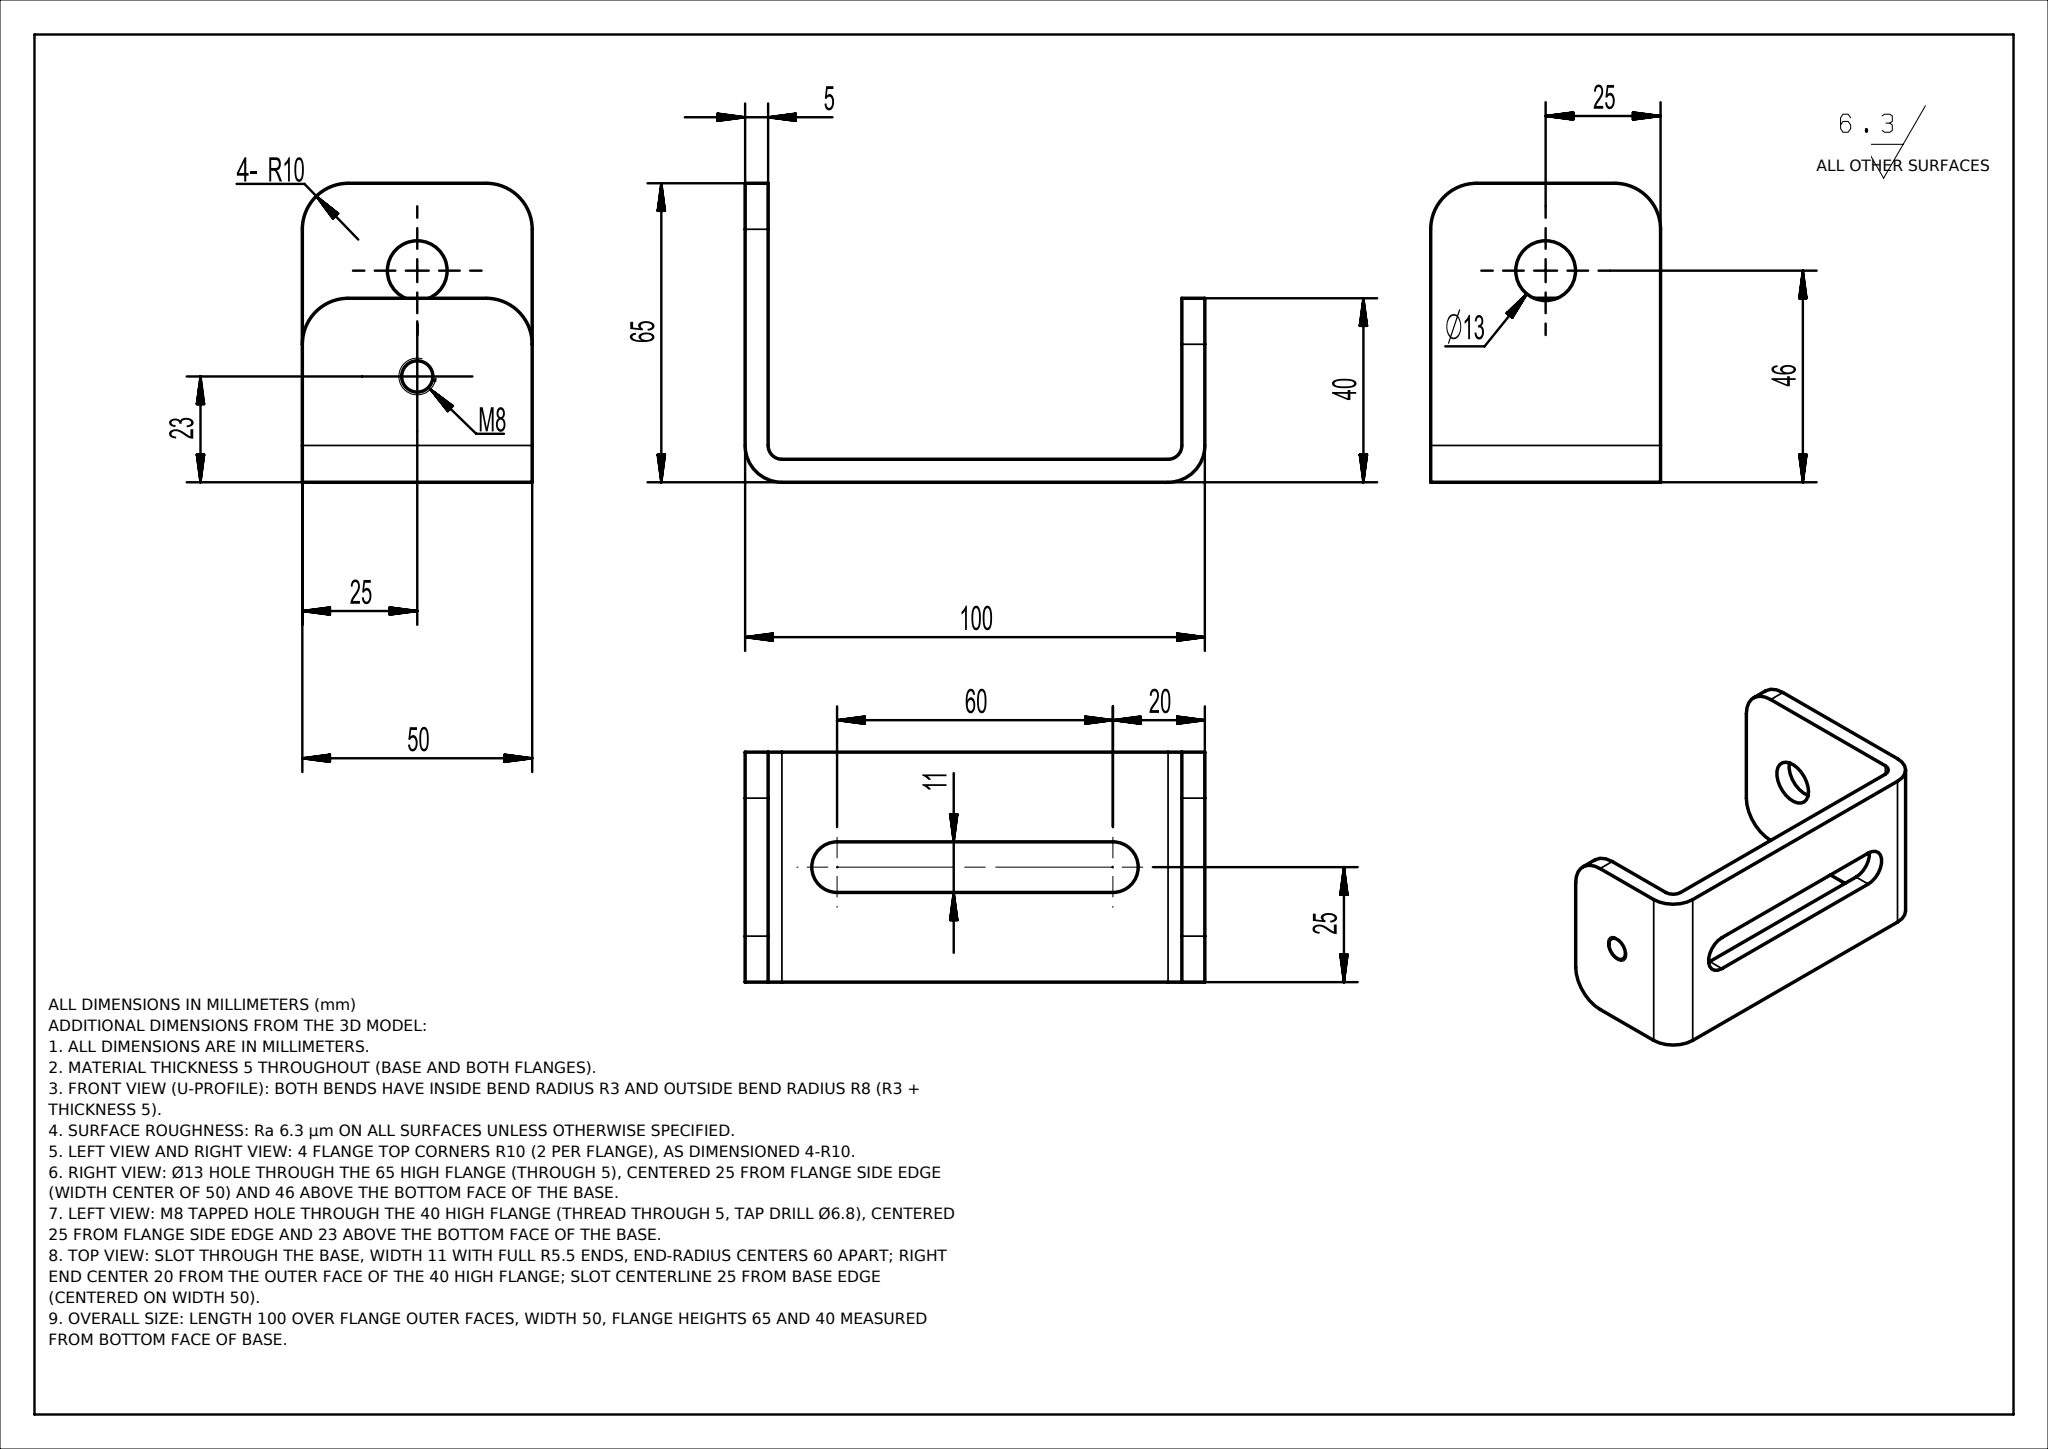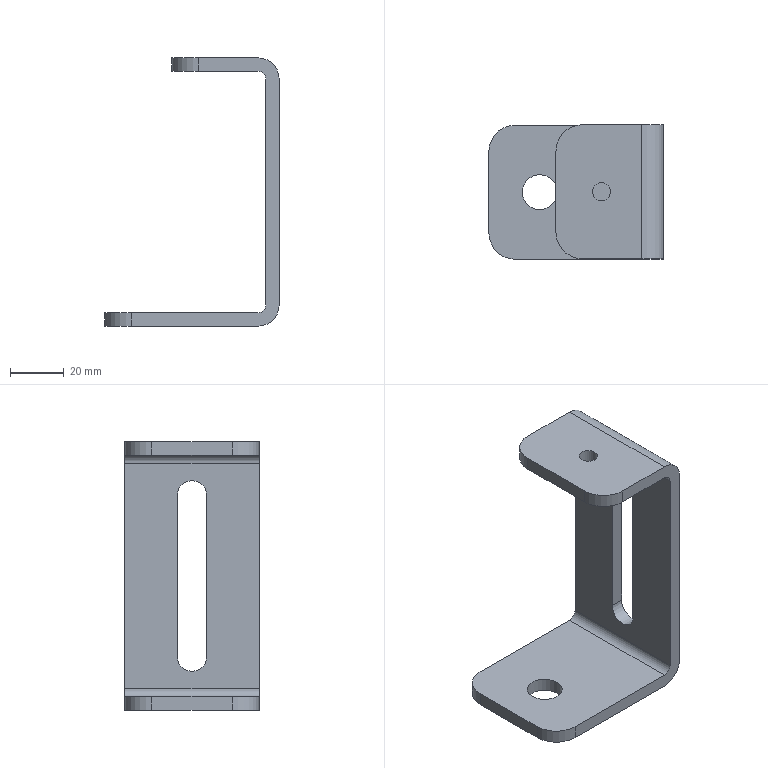Part | NX | mm | 1 solid | 24 faces | box 65 x 50 x 100 mm | volume 42520 mm3 | plane 12 | cylinder 12 | commonest cylinder face diameters 20 x4 6 x2 16 x2 11 x2 6.8 x1 13 x1
STEP:
#1=CARTESIAN_POINT('',(0.,0.,0.));
#2=DIRECTION('',(0.,0.,1.));
#3=DIRECTION('',(1.,0.,0.));
#4=AXIS2_PLACEMENT_3D('',#1,#2,#3);
#5=(LENGTH_UNIT()NAMED_UNIT(*)SI_UNIT(.MILLI.,.METRE.));
#6=UNCERTAINTY_MEASURE_WITH_UNIT(LENGTH_MEASURE(0.00002),#5,'','');
#7=(NAMED_UNIT(*)PLANE_ANGLE_UNIT()SI_UNIT($,.RADIAN.));
#8=PLANE_ANGLE_MEASURE_WITH_UNIT(PLANE_ANGLE_MEASURE(0.01745),#7);
#9=DIMENSIONAL_EXPONENTS(0.,0.,0.,0.,0.,0.,0.);
#10=(CONVERSION_BASED_UNIT('',#8)NAMED_UNIT(#9)PLANE_ANGLE_UNIT());
#11=(NAMED_UNIT(*)SI_UNIT($,.STERADIAN.)SOLID_ANGLE_UNIT());
#12=(GEOMETRIC_REPRESENTATION_CONTEXT(3)GLOBAL_UNCERTAINTY_ASSIGNED_CONTEXT((#6))GLOBAL_UNIT_ASSIGNED_CONTEXT((#5,#10,#11))REPRESENTATION_CONTEXT('',''));
#13=SHAPE_REPRESENTATION('',(#4),#12);
#14=CARTESIAN_POINT('',(10.,0.,5.));
#15=VERTEX_POINT('',#14);
#16=CARTESIAN_POINT('',(57.,0.,5.));
#17=VERTEX_POINT('',#16);
#18=CARTESIAN_POINT('',(0.,0.,5.));
#19=DIRECTION('',(1.,0.,0.));
#20=VECTOR('',#19,1.);
#21=LINE('',#18,#20);
#22=EDGE_CURVE('',#15,#17,#21,.T.);
#23=ORIENTED_EDGE('',*,*,#22,.F.);
#24=CARTESIAN_POINT('',(10.,0.,0.));
#25=VERTEX_POINT('',#24);
#26=CARTESIAN_POINT('',(10.,0.,100.));
#27=DIRECTION('',(0.,0.,-1.));
#28=VECTOR('',#27,1.);
#29=LINE('',#26,#28);
#30=EDGE_CURVE('',#15,#25,#29,.T.);
#31=ORIENTED_EDGE('',*,*,#30,.T.);
#32=CARTESIAN_POINT('',(57.,0.,0.));
#33=VERTEX_POINT('',#32);
#34=CARTESIAN_POINT('',(0.,0.,0.));
#35=DIRECTION('',(1.,0.,0.));
#36=VECTOR('',#35,1.);
#37=LINE('',#34,#36);
#38=EDGE_CURVE('',#25,#33,#37,.T.);
#39=ORIENTED_EDGE('',*,*,#38,.T.);
#40=CARTESIAN_POINT('',(65.,0.,8.));
#41=VERTEX_POINT('',#40);
#42=CARTESIAN_POINT('',(57.,0.,8.));
#43=DIRECTION('',(0.,-1.,0.));
#44=DIRECTION('',(0.,0.,1.));
#45=AXIS2_PLACEMENT_3D('',#42,#43,#44);
#46=CIRCLE('',#45,8.);
#47=EDGE_CURVE('',#33,#41,#46,.T.);
#48=ORIENTED_EDGE('',*,*,#47,.T.);
#49=CARTESIAN_POINT('',(65.,0.,92.));
#50=VERTEX_POINT('',#49);
#51=CARTESIAN_POINT('',(65.,0.,0.));
#52=DIRECTION('',(-0.,0.,1.));
#53=VECTOR('',#52,1.);
#54=LINE('',#51,#53);
#55=EDGE_CURVE('',#41,#50,#54,.T.);
#56=ORIENTED_EDGE('',*,*,#55,.T.);
#57=CARTESIAN_POINT('',(57.,0.,100.));
#58=VERTEX_POINT('',#57);
#59=CARTESIAN_POINT('',(57.,0.,92.));
#60=DIRECTION('',(0.,-1.,0.));
#61=DIRECTION('',(0.,0.,1.));
#62=AXIS2_PLACEMENT_3D('',#59,#60,#61);
#63=CIRCLE('',#62,8.);
#64=EDGE_CURVE('',#50,#58,#63,.T.);
#65=ORIENTED_EDGE('',*,*,#64,.T.);
#66=CARTESIAN_POINT('',(35.,0.,100.));
#67=VERTEX_POINT('',#66);
#68=CARTESIAN_POINT('',(65.,0.,100.));
#69=DIRECTION('',(-1.,0.,0.));
#70=VECTOR('',#69,1.);
#71=LINE('',#68,#70);
#72=EDGE_CURVE('',#58,#67,#71,.T.);
#73=ORIENTED_EDGE('',*,*,#72,.T.);
#74=CARTESIAN_POINT('',(35.,0.,95.));
#75=VERTEX_POINT('',#74);
#76=CARTESIAN_POINT('',(35.,0.,100.));
#77=DIRECTION('',(0.,0.,-1.));
#78=VECTOR('',#77,1.);
#79=LINE('',#76,#78);
#80=EDGE_CURVE('',#67,#75,#79,.T.);
#81=ORIENTED_EDGE('',*,*,#80,.T.);
#82=CARTESIAN_POINT('',(57.,0.,95.));
#83=VERTEX_POINT('',#82);
#84=CARTESIAN_POINT('',(65.,0.,95.));
#85=DIRECTION('',(-1.,0.,0.));
#86=VECTOR('',#85,1.);
#87=LINE('',#84,#86);
#88=EDGE_CURVE('',#83,#75,#87,.T.);
#89=ORIENTED_EDGE('',*,*,#88,.F.);
#90=CARTESIAN_POINT('',(60.,0.,92.));
#91=VERTEX_POINT('',#90);
#92=CARTESIAN_POINT('',(57.,0.,92.));
#93=DIRECTION('',(0.,-1.,0.));
#94=DIRECTION('',(0.,0.,1.));
#95=AXIS2_PLACEMENT_3D('',#92,#93,#94);
#96=CIRCLE('',#95,3.);
#97=EDGE_CURVE('',#91,#83,#96,.T.);
#98=ORIENTED_EDGE('',*,*,#97,.F.);
#99=CARTESIAN_POINT('',(60.,0.,8.));
#100=VERTEX_POINT('',#99);
#101=CARTESIAN_POINT('',(60.,0.,-0.));
#102=DIRECTION('',(-0.,0.,1.));
#103=VECTOR('',#102,1.);
#104=LINE('',#101,#103);
#105=EDGE_CURVE('',#100,#91,#104,.T.);
#106=ORIENTED_EDGE('',*,*,#105,.F.);
#107=CARTESIAN_POINT('',(57.,0.,8.));
#108=DIRECTION('',(0.,-1.,0.));
#109=DIRECTION('',(0.,0.,1.));
#110=AXIS2_PLACEMENT_3D('',#107,#108,#109);
#111=CIRCLE('',#110,3.);
#112=EDGE_CURVE('',#17,#100,#111,.T.);
#113=ORIENTED_EDGE('',*,*,#112,.F.);
#114=EDGE_LOOP('',(#23,#31,#39,#48,#56,#65,#73,#81,#89,#98,#106,#113));
#115=FACE_OUTER_BOUND('',#114,.T.);
#116=CARTESIAN_POINT('',(65.,0.,100.));
#117=DIRECTION('',(0.,-1.,0.));
#118=DIRECTION('',(-1.,0.,0.));
#119=AXIS2_PLACEMENT_3D('',#116,#117,#118);
#120=PLANE('',#119);
#121=ADVANCED_FACE('',(#115),#120,.T.);
#122=CARTESIAN_POINT('',(25.,10.,95.));
#123=VERTEX_POINT('',#122);
#124=CARTESIAN_POINT('',(25.,40.,95.));
#125=VERTEX_POINT('',#124);
#126=CARTESIAN_POINT('',(25.,0.,95.));
#127=DIRECTION('',(0.,1.,0.));
#128=VECTOR('',#127,1.);
#129=LINE('',#126,#128);
#130=EDGE_CURVE('',#123,#125,#129,.T.);
#131=ORIENTED_EDGE('',*,*,#130,.F.);
#132=CARTESIAN_POINT('',(25.,10.,100.));
#133=VERTEX_POINT('',#132);
#134=CARTESIAN_POINT('',(25.,10.,100.));
#135=DIRECTION('',(0.,0.,1.));
#136=VECTOR('',#135,1.);
#137=LINE('',#134,#136);
#138=EDGE_CURVE('',#123,#133,#137,.T.);
#139=ORIENTED_EDGE('',*,*,#138,.T.);
#140=CARTESIAN_POINT('',(25.,40.,100.));
#141=VERTEX_POINT('',#140);
#142=CARTESIAN_POINT('',(25.,0.,100.));
#143=DIRECTION('',(0.,1.,0.));
#144=VECTOR('',#143,1.);
#145=LINE('',#142,#144);
#146=EDGE_CURVE('',#133,#141,#145,.T.);
#147=ORIENTED_EDGE('',*,*,#146,.T.);
#148=CARTESIAN_POINT('',(25.,40.,100.));
#149=DIRECTION('',(0.,0.,-1.));
#150=VECTOR('',#149,1.);
#151=LINE('',#148,#150);
#152=EDGE_CURVE('',#141,#125,#151,.T.);
#153=ORIENTED_EDGE('',*,*,#152,.T.);
#154=EDGE_LOOP('',(#131,#139,#147,#153));
#155=FACE_OUTER_BOUND('',#154,.T.);
#156=CARTESIAN_POINT('',(25.,0.,100.));
#157=DIRECTION('',(-1.,0.,0.));
#158=DIRECTION('',(0.,1.,0.));
#159=AXIS2_PLACEMENT_3D('',#156,#157,#158);
#160=PLANE('',#159);
#161=ADVANCED_FACE('',(#155),#160,.T.);
#162=CARTESIAN_POINT('',(10.,50.,0.));
#163=VERTEX_POINT('',#162);
#164=CARTESIAN_POINT('',(57.,50.,0.));
#165=VERTEX_POINT('',#164);
#166=CARTESIAN_POINT('',(0.,50.,0.));
#167=DIRECTION('',(1.,0.,0.));
#168=VECTOR('',#167,1.);
#169=LINE('',#166,#168);
#170=EDGE_CURVE('',#163,#165,#169,.T.);
#171=ORIENTED_EDGE('',*,*,#170,.F.);
#172=CARTESIAN_POINT('',(10.,50.,5.));
#173=VERTEX_POINT('',#172);
#174=CARTESIAN_POINT('',(10.,50.,0.));
#175=DIRECTION('',(0.,0.,1.));
#176=VECTOR('',#175,1.);
#177=LINE('',#174,#176);
#178=EDGE_CURVE('',#163,#173,#177,.T.);
#179=ORIENTED_EDGE('',*,*,#178,.T.);
#180=CARTESIAN_POINT('',(57.,50.,5.));
#181=VERTEX_POINT('',#180);
#182=CARTESIAN_POINT('',(0.,50.,5.));
#183=DIRECTION('',(1.,0.,0.));
#184=VECTOR('',#183,1.);
#185=LINE('',#182,#184);
#186=EDGE_CURVE('',#173,#181,#185,.T.);
#187=ORIENTED_EDGE('',*,*,#186,.T.);
#188=CARTESIAN_POINT('',(60.,50.,8.));
#189=VERTEX_POINT('',#188);
#190=CARTESIAN_POINT('',(57.,50.,8.));
#191=DIRECTION('',(0.,-1.,0.));
#192=DIRECTION('',(0.,0.,1.));
#193=AXIS2_PLACEMENT_3D('',#190,#191,#192);
#194=CIRCLE('',#193,3.);
#195=EDGE_CURVE('',#181,#189,#194,.T.);
#196=ORIENTED_EDGE('',*,*,#195,.T.);
#197=CARTESIAN_POINT('',(60.,50.,92.));
#198=VERTEX_POINT('',#197);
#199=CARTESIAN_POINT('',(60.,50.,-0.));
#200=DIRECTION('',(-0.,0.,1.));
#201=VECTOR('',#200,1.);
#202=LINE('',#199,#201);
#203=EDGE_CURVE('',#189,#198,#202,.T.);
#204=ORIENTED_EDGE('',*,*,#203,.T.);
#205=CARTESIAN_POINT('',(57.,50.,95.));
#206=VERTEX_POINT('',#205);
#207=CARTESIAN_POINT('',(57.,50.,92.));
#208=DIRECTION('',(0.,-1.,0.));
#209=DIRECTION('',(0.,0.,1.));
#210=AXIS2_PLACEMENT_3D('',#207,#208,#209);
#211=CIRCLE('',#210,3.);
#212=EDGE_CURVE('',#198,#206,#211,.T.);
#213=ORIENTED_EDGE('',*,*,#212,.T.);
#214=CARTESIAN_POINT('',(35.,50.,95.));
#215=VERTEX_POINT('',#214);
#216=CARTESIAN_POINT('',(65.,50.,95.));
#217=DIRECTION('',(-1.,0.,0.));
#218=VECTOR('',#217,1.);
#219=LINE('',#216,#218);
#220=EDGE_CURVE('',#206,#215,#219,.T.);
#221=ORIENTED_EDGE('',*,*,#220,.T.);
#222=CARTESIAN_POINT('',(35.,50.,100.));
#223=VERTEX_POINT('',#222);
#224=CARTESIAN_POINT('',(35.,50.,0.));
#225=DIRECTION('',(0.,0.,1.));
#226=VECTOR('',#225,1.);
#227=LINE('',#224,#226);
#228=EDGE_CURVE('',#215,#223,#227,.T.);
#229=ORIENTED_EDGE('',*,*,#228,.T.);
#230=CARTESIAN_POINT('',(57.,50.,100.));
#231=VERTEX_POINT('',#230);
#232=CARTESIAN_POINT('',(65.,50.,100.));
#233=DIRECTION('',(-1.,0.,0.));
#234=VECTOR('',#233,1.);
#235=LINE('',#232,#234);
#236=EDGE_CURVE('',#231,#223,#235,.T.);
#237=ORIENTED_EDGE('',*,*,#236,.F.);
#238=CARTESIAN_POINT('',(65.,50.,92.));
#239=VERTEX_POINT('',#238);
#240=CARTESIAN_POINT('',(57.,50.,92.));
#241=DIRECTION('',(0.,-1.,0.));
#242=DIRECTION('',(0.,0.,1.));
#243=AXIS2_PLACEMENT_3D('',#240,#241,#242);
#244=CIRCLE('',#243,8.);
#245=EDGE_CURVE('',#239,#231,#244,.T.);
#246=ORIENTED_EDGE('',*,*,#245,.F.);
#247=CARTESIAN_POINT('',(65.,50.,8.));
#248=VERTEX_POINT('',#247);
#249=CARTESIAN_POINT('',(65.,50.,0.));
#250=DIRECTION('',(-0.,0.,1.));
#251=VECTOR('',#250,1.);
#252=LINE('',#249,#251);
#253=EDGE_CURVE('',#248,#239,#252,.T.);
#254=ORIENTED_EDGE('',*,*,#253,.F.);
#255=CARTESIAN_POINT('',(57.,50.,8.));
#256=DIRECTION('',(0.,-1.,0.));
#257=DIRECTION('',(0.,0.,1.));
#258=AXIS2_PLACEMENT_3D('',#255,#256,#257);
#259=CIRCLE('',#258,8.);
#260=EDGE_CURVE('',#165,#248,#259,.T.);
#261=ORIENTED_EDGE('',*,*,#260,.F.);
#262=EDGE_LOOP('',(#171,#179,#187,#196,#204,#213,#221,#229,#237,#246,#254,#261));
#263=FACE_OUTER_BOUND('',#262,.T.);
#264=CARTESIAN_POINT('',(0.,50.,0.));
#265=DIRECTION('',(0.,-1.,0.));
#266=DIRECTION('',(1.,0.,0.));
#267=AXIS2_PLACEMENT_3D('',#264,#265,#266);
#268=PLANE('',#267);
#269=ADVANCED_FACE('',(#263),#268,.F.);
#270=CARTESIAN_POINT('',(0.,10.,0.));
#271=VERTEX_POINT('',#270);
#272=CARTESIAN_POINT('',(0.,40.,0.));
#273=VERTEX_POINT('',#272);
#274=CARTESIAN_POINT('',(0.,0.,0.));
#275=DIRECTION('',(0.,1.,0.));
#276=VECTOR('',#275,1.);
#277=LINE('',#274,#276);
#278=EDGE_CURVE('',#271,#273,#277,.T.);
#279=ORIENTED_EDGE('',*,*,#278,.F.);
#280=CARTESIAN_POINT('',(0.,10.,5.));
#281=VERTEX_POINT('',#280);
#282=CARTESIAN_POINT('',(0.,10.,0.));
#283=DIRECTION('',(0.,0.,1.));
#284=VECTOR('',#283,1.);
#285=LINE('',#282,#284);
#286=EDGE_CURVE('',#271,#281,#285,.T.);
#287=ORIENTED_EDGE('',*,*,#286,.T.);
#288=CARTESIAN_POINT('',(0.,40.,5.));
#289=VERTEX_POINT('',#288);
#290=CARTESIAN_POINT('',(0.,0.,5.));
#291=DIRECTION('',(0.,1.,0.));
#292=VECTOR('',#291,1.);
#293=LINE('',#290,#292);
#294=EDGE_CURVE('',#281,#289,#293,.T.);
#295=ORIENTED_EDGE('',*,*,#294,.T.);
#296=CARTESIAN_POINT('',(0.,40.,0.));
#297=DIRECTION('',(0.,0.,-1.));
#298=VECTOR('',#297,1.);
#299=LINE('',#296,#298);
#300=EDGE_CURVE('',#289,#273,#299,.T.);
#301=ORIENTED_EDGE('',*,*,#300,.T.);
#302=EDGE_LOOP('',(#279,#287,#295,#301));
#303=FACE_OUTER_BOUND('',#302,.T.);
#304=CARTESIAN_POINT('',(0.,0.,0.));
#305=DIRECTION('',(1.,0.,0.));
#306=DIRECTION('',(0.,1.,0.));
#307=AXIS2_PLACEMENT_3D('',#304,#305,#306);
#308=PLANE('',#307);
#309=ADVANCED_FACE('',(#303),#308,.F.);
#310=CARTESIAN_POINT('',(25.5,25.,5.));
#311=VERTEX_POINT('',#310);
#312=CARTESIAN_POINT('',(19.,25.,5.));
#313=DIRECTION('',(0.,0.,-1.));
#314=DIRECTION('',(1.,0.,0.));
#315=AXIS2_PLACEMENT_3D('',#312,#313,#314);
#316=CIRCLE('',#315,6.5);
#317=EDGE_CURVE('',#311,#311,#316,.T.);
#318=ORIENTED_EDGE('',*,*,#317,.T.);
#319=EDGE_LOOP('',(#318));
#320=FACE_BOUND('',#319,.T.);
#321=ORIENTED_EDGE('',*,*,#294,.F.);
#322=CARTESIAN_POINT('',(10.,10.,5.));
#323=DIRECTION('',(0.,0.,1.));
#324=DIRECTION('',(1.,0.,0.));
#325=AXIS2_PLACEMENT_3D('',#322,#323,#324);
#326=CIRCLE('',#325,10.);
#327=EDGE_CURVE('',#281,#15,#326,.T.);
#328=ORIENTED_EDGE('',*,*,#327,.T.);
#329=ORIENTED_EDGE('',*,*,#22,.T.);
#330=CARTESIAN_POINT('',(57.,0.,5.));
#331=DIRECTION('',(0.,1.,0.));
#332=VECTOR('',#331,1.);
#333=LINE('',#330,#332);
#334=EDGE_CURVE('',#17,#181,#333,.T.);
#335=ORIENTED_EDGE('',*,*,#334,.T.);
#336=ORIENTED_EDGE('',*,*,#186,.F.);
#337=CARTESIAN_POINT('',(10.,40.,5.));
#338=DIRECTION('',(0.,0.,1.));
#339=DIRECTION('',(1.,0.,0.));
#340=AXIS2_PLACEMENT_3D('',#337,#338,#339);
#341=CIRCLE('',#340,10.);
#342=EDGE_CURVE('',#173,#289,#341,.T.);
#343=ORIENTED_EDGE('',*,*,#342,.T.);
#344=EDGE_LOOP('',(#321,#328,#329,#335,#336,#343));
#345=FACE_BOUND('',#344,.T.);
#346=CARTESIAN_POINT('',(0.,0.,5.));
#347=DIRECTION('',(0.,0.,1.));
#348=DIRECTION('',(1.,0.,0.));
#349=AXIS2_PLACEMENT_3D('',#346,#347,#348);
#350=PLANE('',#349);
#351=ADVANCED_FACE('',(#320,#345),#350,.T.);
#352=ORIENTED_EDGE('',*,*,#195,.F.);
#353=ORIENTED_EDGE('',*,*,#334,.F.);
#354=ORIENTED_EDGE('',*,*,#112,.T.);
#355=CARTESIAN_POINT('',(60.,0.,8.));
#356=DIRECTION('',(0.,1.,0.));
#357=VECTOR('',#356,1.);
#358=LINE('',#355,#357);
#359=EDGE_CURVE('',#100,#189,#358,.T.);
#360=ORIENTED_EDGE('',*,*,#359,.T.);
#361=EDGE_LOOP('',(#352,#353,#354,#360));
#362=FACE_OUTER_BOUND('',#361,.T.);
#363=CARTESIAN_POINT('',(57.,0.,8.));
#364=DIRECTION('',(0.,1.,0.));
#365=DIRECTION('',(0.,0.,1.));
#366=AXIS2_PLACEMENT_3D('',#363,#364,#365);
#367=CYLINDRICAL_SURFACE('',#366,3.);
#368=ADVANCED_FACE('',(#362),#367,.F.);
#369=CARTESIAN_POINT('',(60.,30.5,80.));
#370=VERTEX_POINT('',#369);
#371=CARTESIAN_POINT('',(60.,19.5,80.));
#372=VERTEX_POINT('',#371);
#373=CARTESIAN_POINT('',(60.,25.,80.));
#374=DIRECTION('',(1.,0.,0.));
#375=DIRECTION('',(0.,0.,1.));
#376=AXIS2_PLACEMENT_3D('',#373,#374,#375);
#377=CIRCLE('',#376,5.5);
#378=EDGE_CURVE('',#370,#372,#377,.T.);
#379=ORIENTED_EDGE('',*,*,#378,.T.);
#380=CARTESIAN_POINT('',(60.,19.5,20.));
#381=VERTEX_POINT('',#380);
#382=CARTESIAN_POINT('',(60.,19.5,-0.));
#383=DIRECTION('',(0.,0.,-1.));
#384=VECTOR('',#383,1.);
#385=LINE('',#382,#384);
#386=EDGE_CURVE('',#372,#381,#385,.T.);
#387=ORIENTED_EDGE('',*,*,#386,.T.);
#388=CARTESIAN_POINT('',(60.,30.5,20.));
#389=VERTEX_POINT('',#388);
#390=CARTESIAN_POINT('',(60.,25.,20.));
#391=DIRECTION('',(1.,0.,0.));
#392=DIRECTION('',(0.,0.,1.));
#393=AXIS2_PLACEMENT_3D('',#390,#391,#392);
#394=CIRCLE('',#393,5.5);
#395=EDGE_CURVE('',#381,#389,#394,.T.);
#396=ORIENTED_EDGE('',*,*,#395,.T.);
#397=CARTESIAN_POINT('',(60.,30.5,-0.));
#398=DIRECTION('',(-0.,0.,1.));
#399=VECTOR('',#398,1.);
#400=LINE('',#397,#399);
#401=EDGE_CURVE('',#389,#370,#400,.T.);
#402=ORIENTED_EDGE('',*,*,#401,.T.);
#403=EDGE_LOOP('',(#379,#387,#396,#402));
#404=FACE_BOUND('',#403,.T.);
#405=ORIENTED_EDGE('',*,*,#203,.F.);
#406=ORIENTED_EDGE('',*,*,#359,.F.);
#407=ORIENTED_EDGE('',*,*,#105,.T.);
#408=CARTESIAN_POINT('',(60.,0.,92.));
#409=DIRECTION('',(0.,1.,0.));
#410=VECTOR('',#409,1.);
#411=LINE('',#408,#410);
#412=EDGE_CURVE('',#91,#198,#411,.T.);
#413=ORIENTED_EDGE('',*,*,#412,.T.);
#414=EDGE_LOOP('',(#405,#406,#407,#413));
#415=FACE_BOUND('',#414,.T.);
#416=CARTESIAN_POINT('',(60.,0.,-0.));
#417=DIRECTION('',(-1.,0.,-0.));
#418=DIRECTION('',(-0.,0.,1.));
#419=AXIS2_PLACEMENT_3D('',#416,#417,#418);
#420=PLANE('',#419);
#421=ADVANCED_FACE('',(#404,#415),#420,.T.);
#422=ORIENTED_EDGE('',*,*,#212,.F.);
#423=ORIENTED_EDGE('',*,*,#412,.F.);
#424=ORIENTED_EDGE('',*,*,#97,.T.);
#425=CARTESIAN_POINT('',(57.,0.,95.));
#426=DIRECTION('',(0.,1.,0.));
#427=VECTOR('',#426,1.);
#428=LINE('',#425,#427);
#429=EDGE_CURVE('',#83,#206,#428,.T.);
#430=ORIENTED_EDGE('',*,*,#429,.T.);
#431=EDGE_LOOP('',(#422,#423,#424,#430));
#432=FACE_OUTER_BOUND('',#431,.T.);
#433=CARTESIAN_POINT('',(57.,0.,92.));
#434=DIRECTION('',(0.,1.,0.));
#435=DIRECTION('',(0.,0.,1.));
#436=AXIS2_PLACEMENT_3D('',#433,#434,#435);
#437=CYLINDRICAL_SURFACE('',#436,3.);
#438=ADVANCED_FACE('',(#432),#437,.F.);
#439=CARTESIAN_POINT('',(38.6,25.,95.));
#440=VERTEX_POINT('',#439);
#441=CARTESIAN_POINT('',(42.,25.,95.));
#442=DIRECTION('',(0.,0.,-1.));
#443=DIRECTION('',(-1.,0.,0.));
#444=AXIS2_PLACEMENT_3D('',#441,#442,#443);
#445=CIRCLE('',#444,3.4);
#446=EDGE_CURVE('',#440,#440,#445,.T.);
#447=ORIENTED_EDGE('',*,*,#446,.F.);
#448=EDGE_LOOP('',(#447));
#449=FACE_BOUND('',#448,.T.);
#450=ORIENTED_EDGE('',*,*,#88,.T.);
#451=CARTESIAN_POINT('',(35.,10.,95.));
#452=DIRECTION('',(0.,0.,-1.));
#453=DIRECTION('',(-1.,0.,0.));
#454=AXIS2_PLACEMENT_3D('',#451,#452,#453);
#455=CIRCLE('',#454,10.);
#456=EDGE_CURVE('',#75,#123,#455,.T.);
#457=ORIENTED_EDGE('',*,*,#456,.T.);
#458=ORIENTED_EDGE('',*,*,#130,.T.);
#459=CARTESIAN_POINT('',(35.,40.,95.));
#460=DIRECTION('',(0.,0.,-1.));
#461=DIRECTION('',(-1.,0.,0.));
#462=AXIS2_PLACEMENT_3D('',#459,#460,#461);
#463=CIRCLE('',#462,10.);
#464=EDGE_CURVE('',#125,#215,#463,.T.);
#465=ORIENTED_EDGE('',*,*,#464,.T.);
#466=ORIENTED_EDGE('',*,*,#220,.F.);
#467=ORIENTED_EDGE('',*,*,#429,.F.);
#468=EDGE_LOOP('',(#450,#457,#458,#465,#466,#467));
#469=FACE_BOUND('',#468,.T.);
#470=CARTESIAN_POINT('',(65.,0.,95.));
#471=DIRECTION('',(0.,0.,-1.));
#472=DIRECTION('',(-1.,0.,0.));
#473=AXIS2_PLACEMENT_3D('',#470,#471,#472);
#474=PLANE('',#473);
#475=ADVANCED_FACE('',(#449,#469),#474,.T.);
#476=CARTESIAN_POINT('',(25.5,25.,0.));
#477=VERTEX_POINT('',#476);
#478=CARTESIAN_POINT('',(19.,25.,0.));
#479=DIRECTION('',(0.,0.,-1.));
#480=DIRECTION('',(1.,0.,0.));
#481=AXIS2_PLACEMENT_3D('',#478,#479,#480);
#482=CIRCLE('',#481,6.5);
#483=EDGE_CURVE('',#477,#477,#482,.T.);
#484=ORIENTED_EDGE('',*,*,#483,.F.);
#485=EDGE_LOOP('',(#484));
#486=FACE_BOUND('',#485,.T.);
#487=ORIENTED_EDGE('',*,*,#38,.F.);
#488=CARTESIAN_POINT('',(10.,10.,0.));
#489=DIRECTION('',(0.,0.,-1.));
#490=DIRECTION('',(1.,0.,0.));
#491=AXIS2_PLACEMENT_3D('',#488,#489,#490);
#492=CIRCLE('',#491,10.);
#493=EDGE_CURVE('',#25,#271,#492,.T.);
#494=ORIENTED_EDGE('',*,*,#493,.T.);
#495=ORIENTED_EDGE('',*,*,#278,.T.);
#496=CARTESIAN_POINT('',(10.,40.,0.));
#497=DIRECTION('',(0.,0.,-1.));
#498=DIRECTION('',(1.,0.,0.));
#499=AXIS2_PLACEMENT_3D('',#496,#497,#498);
#500=CIRCLE('',#499,10.);
#501=EDGE_CURVE('',#273,#163,#500,.T.);
#502=ORIENTED_EDGE('',*,*,#501,.T.);
#503=ORIENTED_EDGE('',*,*,#170,.T.);
#504=CARTESIAN_POINT('',(57.,0.,0.));
#505=DIRECTION('',(0.,1.,0.));
#506=VECTOR('',#505,1.);
#507=LINE('',#504,#506);
#508=EDGE_CURVE('',#33,#165,#507,.T.);
#509=ORIENTED_EDGE('',*,*,#508,.F.);
#510=EDGE_LOOP('',(#487,#494,#495,#502,#503,#509));
#511=FACE_BOUND('',#510,.T.);
#512=CARTESIAN_POINT('',(0.,0.,0.));
#513=DIRECTION('',(0.,0.,1.));
#514=DIRECTION('',(1.,0.,0.));
#515=AXIS2_PLACEMENT_3D('',#512,#513,#514);
#516=PLANE('',#515);
#517=ADVANCED_FACE('',(#486,#511),#516,.F.);
#518=ORIENTED_EDGE('',*,*,#260,.T.);
#519=CARTESIAN_POINT('',(65.,0.,8.));
#520=DIRECTION('',(0.,1.,0.));
#521=VECTOR('',#520,1.);
#522=LINE('',#519,#521);
#523=EDGE_CURVE('',#41,#248,#522,.T.);
#524=ORIENTED_EDGE('',*,*,#523,.F.);
#525=ORIENTED_EDGE('',*,*,#47,.F.);
#526=ORIENTED_EDGE('',*,*,#508,.T.);
#527=EDGE_LOOP('',(#518,#524,#525,#526));
#528=FACE_OUTER_BOUND('',#527,.T.);
#529=CARTESIAN_POINT('',(57.,0.,8.));
#530=DIRECTION('',(0.,1.,0.));
#531=DIRECTION('',(0.,0.,1.));
#532=AXIS2_PLACEMENT_3D('',#529,#530,#531);
#533=CYLINDRICAL_SURFACE('',#532,8.);
#534=ADVANCED_FACE('',(#528),#533,.T.);
#535=CARTESIAN_POINT('',(65.,19.5,80.));
#536=VERTEX_POINT('',#535);
#537=CARTESIAN_POINT('',(65.,19.5,20.));
#538=VERTEX_POINT('',#537);
#539=CARTESIAN_POINT('',(65.,19.5,0.));
#540=DIRECTION('',(0.,0.,-1.));
#541=VECTOR('',#540,1.);
#542=LINE('',#539,#541);
#543=EDGE_CURVE('',#536,#538,#542,.T.);
#544=ORIENTED_EDGE('',*,*,#543,.F.);
#545=CARTESIAN_POINT('',(65.,30.5,80.));
#546=VERTEX_POINT('',#545);
#547=CARTESIAN_POINT('',(65.,25.,80.));
#548=DIRECTION('',(1.,0.,0.));
#549=DIRECTION('',(0.,0.,1.));
#550=AXIS2_PLACEMENT_3D('',#547,#548,#549);
#551=CIRCLE('',#550,5.5);
#552=EDGE_CURVE('',#546,#536,#551,.T.);
#553=ORIENTED_EDGE('',*,*,#552,.F.);
#554=CARTESIAN_POINT('',(65.,30.5,20.));
#555=VERTEX_POINT('',#554);
#556=CARTESIAN_POINT('',(65.,30.5,0.));
#557=DIRECTION('',(-0.,0.,1.));
#558=VECTOR('',#557,1.);
#559=LINE('',#556,#558);
#560=EDGE_CURVE('',#555,#546,#559,.T.);
#561=ORIENTED_EDGE('',*,*,#560,.F.);
#562=CARTESIAN_POINT('',(65.,25.,20.));
#563=DIRECTION('',(1.,0.,0.));
#564=DIRECTION('',(0.,0.,1.));
#565=AXIS2_PLACEMENT_3D('',#562,#563,#564);
#566=CIRCLE('',#565,5.5);
#567=EDGE_CURVE('',#538,#555,#566,.T.);
#568=ORIENTED_EDGE('',*,*,#567,.F.);
#569=EDGE_LOOP('',(#544,#553,#561,#568));
#570=FACE_BOUND('',#569,.T.);
#571=ORIENTED_EDGE('',*,*,#253,.T.);
#572=CARTESIAN_POINT('',(65.,0.,92.));
#573=DIRECTION('',(0.,1.,0.));
#574=VECTOR('',#573,1.);
#575=LINE('',#572,#574);
#576=EDGE_CURVE('',#50,#239,#575,.T.);
#577=ORIENTED_EDGE('',*,*,#576,.F.);
#578=ORIENTED_EDGE('',*,*,#55,.F.);
#579=ORIENTED_EDGE('',*,*,#523,.T.);
#580=EDGE_LOOP('',(#571,#577,#578,#579));
#581=FACE_BOUND('',#580,.T.);
#582=CARTESIAN_POINT('',(65.,0.,0.));
#583=DIRECTION('',(-1.,0.,-0.));
#584=DIRECTION('',(-0.,0.,1.));
#585=AXIS2_PLACEMENT_3D('',#582,#583,#584);
#586=PLANE('',#585);
#587=ADVANCED_FACE('',(#570,#581),#586,.F.);
#588=ORIENTED_EDGE('',*,*,#245,.T.);
#589=CARTESIAN_POINT('',(57.,0.,100.));
#590=DIRECTION('',(0.,1.,0.));
#591=VECTOR('',#590,1.);
#592=LINE('',#589,#591);
#593=EDGE_CURVE('',#58,#231,#592,.T.);
#594=ORIENTED_EDGE('',*,*,#593,.F.);
#595=ORIENTED_EDGE('',*,*,#64,.F.);
#596=ORIENTED_EDGE('',*,*,#576,.T.);
#597=EDGE_LOOP('',(#588,#594,#595,#596));
#598=FACE_OUTER_BOUND('',#597,.T.);
#599=CARTESIAN_POINT('',(57.,0.,92.));
#600=DIRECTION('',(0.,1.,0.));
#601=DIRECTION('',(0.,0.,1.));
#602=AXIS2_PLACEMENT_3D('',#599,#600,#601);
#603=CYLINDRICAL_SURFACE('',#602,8.);
#604=ADVANCED_FACE('',(#598),#603,.T.);
#605=CARTESIAN_POINT('',(38.6,25.,100.));
#606=VERTEX_POINT('',#605);
#607=CARTESIAN_POINT('',(42.,25.,100.));
#608=DIRECTION('',(0.,0.,-1.));
#609=DIRECTION('',(-1.,0.,0.));
#610=AXIS2_PLACEMENT_3D('',#607,#608,#609);
#611=CIRCLE('',#610,3.4);
#612=EDGE_CURVE('',#606,#606,#611,.T.);
#613=ORIENTED_EDGE('',*,*,#612,.T.);
#614=EDGE_LOOP('',(#613));
#615=FACE_BOUND('',#614,.T.);
#616=ORIENTED_EDGE('',*,*,#146,.F.);
#617=CARTESIAN_POINT('',(35.,10.,100.));
#618=DIRECTION('',(0.,0.,1.));
#619=DIRECTION('',(-1.,0.,0.));
#620=AXIS2_PLACEMENT_3D('',#617,#618,#619);
#621=CIRCLE('',#620,10.);
#622=EDGE_CURVE('',#133,#67,#621,.T.);
#623=ORIENTED_EDGE('',*,*,#622,.T.);
#624=ORIENTED_EDGE('',*,*,#72,.F.);
#625=ORIENTED_EDGE('',*,*,#593,.T.);
#626=ORIENTED_EDGE('',*,*,#236,.T.);
#627=CARTESIAN_POINT('',(35.,40.,100.));
#628=DIRECTION('',(0.,0.,1.));
#629=DIRECTION('',(-1.,0.,0.));
#630=AXIS2_PLACEMENT_3D('',#627,#628,#629);
#631=CIRCLE('',#630,10.);
#632=EDGE_CURVE('',#223,#141,#631,.T.);
#633=ORIENTED_EDGE('',*,*,#632,.T.);
#634=EDGE_LOOP('',(#616,#623,#624,#625,#626,#633));
#635=FACE_BOUND('',#634,.T.);
#636=CARTESIAN_POINT('',(65.,0.,100.));
#637=DIRECTION('',(0.,0.,-1.));
#638=DIRECTION('',(-1.,0.,0.));
#639=AXIS2_PLACEMENT_3D('',#636,#637,#638);
#640=PLANE('',#639);
#641=ADVANCED_FACE('',(#615,#635),#640,.F.);
#642=ORIENTED_EDGE('',*,*,#493,.F.);
#643=ORIENTED_EDGE('',*,*,#30,.F.);
#644=ORIENTED_EDGE('',*,*,#327,.F.);
#645=ORIENTED_EDGE('',*,*,#286,.F.);
#646=EDGE_LOOP('',(#642,#643,#644,#645));
#647=FACE_OUTER_BOUND('',#646,.T.);
#648=CARTESIAN_POINT('',(10.,10.,0.));
#649=DIRECTION('',(0.,0.,-1.));
#650=DIRECTION('',(-1.,0.,0.));
#651=AXIS2_PLACEMENT_3D('',#648,#649,#650);
#652=CYLINDRICAL_SURFACE('',#651,10.);
#653=ADVANCED_FACE('',(#647),#652,.T.);
#654=ORIENTED_EDGE('',*,*,#501,.F.);
#655=ORIENTED_EDGE('',*,*,#300,.F.);
#656=ORIENTED_EDGE('',*,*,#342,.F.);
#657=ORIENTED_EDGE('',*,*,#178,.F.);
#658=EDGE_LOOP('',(#654,#655,#656,#657));
#659=FACE_OUTER_BOUND('',#658,.T.);
#660=CARTESIAN_POINT('',(10.,40.,0.));
#661=DIRECTION('',(0.,0.,1.));
#662=DIRECTION('',(1.,0.,0.));
#663=AXIS2_PLACEMENT_3D('',#660,#661,#662);
#664=CYLINDRICAL_SURFACE('',#663,10.);
#665=ADVANCED_FACE('',(#659),#664,.T.);
#666=ORIENTED_EDGE('',*,*,#622,.F.);
#667=ORIENTED_EDGE('',*,*,#138,.F.);
#668=ORIENTED_EDGE('',*,*,#456,.F.);
#669=ORIENTED_EDGE('',*,*,#80,.F.);
#670=EDGE_LOOP('',(#666,#667,#668,#669));
#671=FACE_OUTER_BOUND('',#670,.T.);
#672=CARTESIAN_POINT('',(35.,10.,100.));
#673=DIRECTION('',(0.,0.,-1.));
#674=DIRECTION('',(-1.,0.,0.));
#675=AXIS2_PLACEMENT_3D('',#672,#673,#674);
#676=CYLINDRICAL_SURFACE('',#675,10.);
#677=ADVANCED_FACE('',(#671),#676,.T.);
#678=ORIENTED_EDGE('',*,*,#632,.F.);
#679=ORIENTED_EDGE('',*,*,#228,.F.);
#680=ORIENTED_EDGE('',*,*,#464,.F.);
#681=ORIENTED_EDGE('',*,*,#152,.F.);
#682=EDGE_LOOP('',(#678,#679,#680,#681));
#683=FACE_OUTER_BOUND('',#682,.T.);
#684=CARTESIAN_POINT('',(35.,40.,100.));
#685=DIRECTION('',(0.,0.,1.));
#686=DIRECTION('',(1.,0.,0.));
#687=AXIS2_PLACEMENT_3D('',#684,#685,#686);
#688=CYLINDRICAL_SURFACE('',#687,10.);
#689=ADVANCED_FACE('',(#683),#688,.T.);
#690=CARTESIAN_POINT('',(52.,19.5,80.));
#691=DIRECTION('',(-1.,0.,0.));
#692=VECTOR('',#691,1.);
#693=LINE('',#690,#692);
#694=EDGE_CURVE('',#536,#372,#693,.T.);
#695=ORIENTED_EDGE('',*,*,#694,.F.);
#696=ORIENTED_EDGE('',*,*,#543,.T.);
#697=CARTESIAN_POINT('',(52.,19.5,20.));
#698=DIRECTION('',(-1.,0.,0.));
#699=VECTOR('',#698,1.);
#700=LINE('',#697,#699);
#701=EDGE_CURVE('',#538,#381,#700,.T.);
#702=ORIENTED_EDGE('',*,*,#701,.T.);
#703=ORIENTED_EDGE('',*,*,#386,.F.);
#704=EDGE_LOOP('',(#695,#696,#702,#703));
#705=FACE_OUTER_BOUND('',#704,.T.);
#706=CARTESIAN_POINT('',(52.,19.5,20.));
#707=DIRECTION('',(0.,1.,0.));
#708=DIRECTION('',(0.,0.,1.));
#709=AXIS2_PLACEMENT_3D('',#706,#707,#708);
#710=PLANE('',#709);
#711=ADVANCED_FACE('',(#705),#710,.T.);
#712=CARTESIAN_POINT('',(52.,30.5,80.));
#713=DIRECTION('',(-1.,0.,0.));
#714=VECTOR('',#713,1.);
#715=LINE('',#712,#714);
#716=EDGE_CURVE('',#546,#370,#715,.T.);
#717=ORIENTED_EDGE('',*,*,#716,.F.);
#718=ORIENTED_EDGE('',*,*,#552,.T.);
#719=ORIENTED_EDGE('',*,*,#694,.T.);
#720=ORIENTED_EDGE('',*,*,#378,.F.);
#721=EDGE_LOOP('',(#717,#718,#719,#720));
#722=FACE_OUTER_BOUND('',#721,.T.);
#723=CARTESIAN_POINT('',(52.,25.,80.));
#724=DIRECTION('',(1.,0.,0.));
#725=DIRECTION('',(0.,0.,-1.));
#726=AXIS2_PLACEMENT_3D('',#723,#724,#725);
#727=CYLINDRICAL_SURFACE('',#726,5.5);
#728=ADVANCED_FACE('',(#722),#727,.F.);
#729=CARTESIAN_POINT('',(52.,30.5,20.));
#730=DIRECTION('',(-1.,0.,0.));
#731=VECTOR('',#730,1.);
#732=LINE('',#729,#731);
#733=EDGE_CURVE('',#555,#389,#732,.T.);
#734=ORIENTED_EDGE('',*,*,#733,.F.);
#735=ORIENTED_EDGE('',*,*,#560,.T.);
#736=ORIENTED_EDGE('',*,*,#716,.T.);
#737=ORIENTED_EDGE('',*,*,#401,.F.);
#738=EDGE_LOOP('',(#734,#735,#736,#737));
#739=FACE_OUTER_BOUND('',#738,.T.);
#740=CARTESIAN_POINT('',(52.,30.5,80.));
#741=DIRECTION('',(0.,-1.,0.));
#742=DIRECTION('',(0.,0.,-1.));
#743=AXIS2_PLACEMENT_3D('',#740,#741,#742);
#744=PLANE('',#743);
#745=ADVANCED_FACE('',(#739),#744,.T.);
#746=ORIENTED_EDGE('',*,*,#701,.F.);
#747=ORIENTED_EDGE('',*,*,#567,.T.);
#748=ORIENTED_EDGE('',*,*,#733,.T.);
#749=ORIENTED_EDGE('',*,*,#395,.F.);
#750=EDGE_LOOP('',(#746,#747,#748,#749));
#751=FACE_OUTER_BOUND('',#750,.T.);
#752=CARTESIAN_POINT('',(52.,25.,20.));
#753=DIRECTION('',(1.,0.,0.));
#754=DIRECTION('',(0.,0.,-1.));
#755=AXIS2_PLACEMENT_3D('',#752,#753,#754);
#756=CYLINDRICAL_SURFACE('',#755,5.5);
#757=ADVANCED_FACE('',(#751),#756,.F.);
#758=ORIENTED_EDGE('',*,*,#446,.T.);
#759=EDGE_LOOP('',(#758));
#760=FACE_BOUND('',#759,.T.);
#761=ORIENTED_EDGE('',*,*,#612,.F.);
#762=EDGE_LOOP('',(#761));
#763=FACE_BOUND('',#762,.T.);
#764=CARTESIAN_POINT('',(42.,25.,100.));
#765=DIRECTION('',(0.,0.,-1.));
#766=DIRECTION('',(-1.,0.,0.));
#767=AXIS2_PLACEMENT_3D('',#764,#765,#766);
#768=CYLINDRICAL_SURFACE('',#767,3.4);
#769=ADVANCED_FACE('',(#760,#763),#768,.F.);
#770=ORIENTED_EDGE('',*,*,#317,.F.);
#771=EDGE_LOOP('',(#770));
#772=FACE_BOUND('',#771,.T.);
#773=ORIENTED_EDGE('',*,*,#483,.T.);
#774=EDGE_LOOP('',(#773));
#775=FACE_BOUND('',#774,.T.);
#776=CARTESIAN_POINT('',(19.,25.,13.));
#777=DIRECTION('',(0.,0.,-1.));
#778=DIRECTION('',(-1.,0.,0.));
#779=AXIS2_PLACEMENT_3D('',#776,#777,#778);
#780=CYLINDRICAL_SURFACE('',#779,6.5);
#781=ADVANCED_FACE('',(#772,#775),#780,.F.);
#782=CLOSED_SHELL('',(#121,#161,#269,#309,#351,#368,#421,#438,#475,#517,#534,#587,#604,#641,#653,#665,#677,#689,#711,#728,#745,#757,#769,#781));
#783=MANIFOLD_SOLID_BREP('',#782);
#784=ADVANCED_BREP_SHAPE_REPRESENTATION('',(#783),#12);
#785=SHAPE_REPRESENTATION_RELATIONSHIP('','',#13,#784);
#786=PRESENTATION_LAYER_ASSIGNMENT('','',(#783));
#787=COLOUR_RGB('',0.8,0.8,0.8);
#788=FILL_AREA_STYLE_COLOUR('',#787);
#789=FILL_AREA_STYLE('',(#788));
#790=SURFACE_STYLE_FILL_AREA(#789);
#791=SURFACE_SIDE_STYLE('',(#790));
#792=SURFACE_STYLE_USAGE(.BOTH.,#791);
#793=PRESENTATION_STYLE_ASSIGNMENT((#792));
#794=STYLED_ITEM('',(#793),#783);
#795=MECHANICAL_DESIGN_GEOMETRIC_PRESENTATION_REPRESENTATION('',(#794),#12);